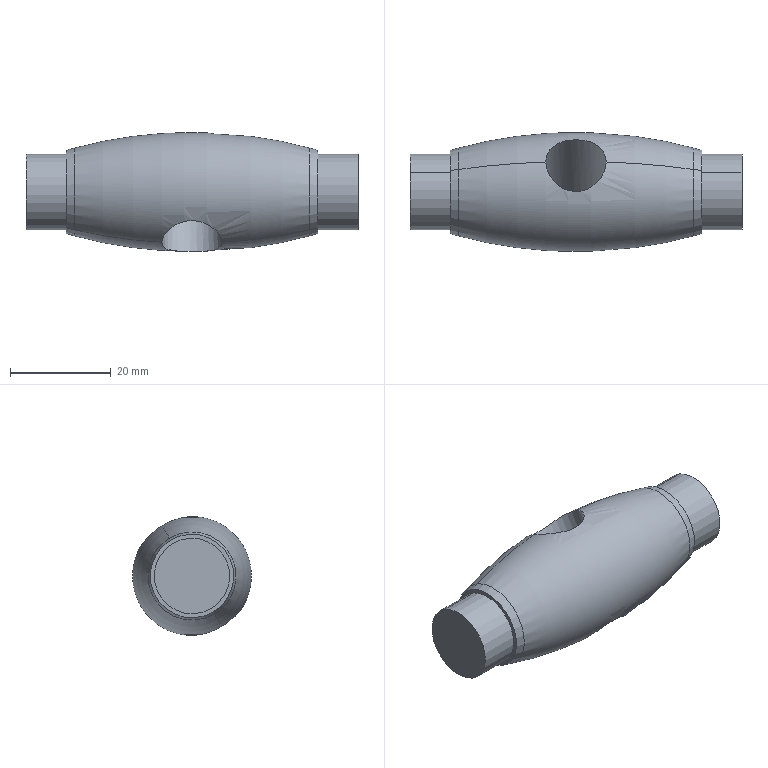Component | SolidWorks | ShaftStop-1 | 1 solid | 16 faces | volume 18258 mm3 | cylinder 6 | cone 4 | plane 4 | torus 2 | commonest cylinder face diameters 15 x4 12 x2
build123d program:
from build123d import *

# Parameters (mm, degrees)
SKETCH1_R           = 15
BOSS_EXTRUDE1_DEPTH = 25
BOSS_EXTRUDE1_TAPER = 15
SKETCH2_R           = 7.5
BOSS_EXTRUDE2_DEPTH = 8
FILLET1_R           = 90
SKETCH3_R           = 6
CUT_EXTRUDE1_DEPTH  = 16.5


with BuildPart() as part:
    # Sketch1 → Boss-Extrude1 (new body)
    with BuildSketch(Plane.XY):
        Circle(SKETCH1_R)
    boss_extrude1 = extrude(amount=BOSS_EXTRUDE1_DEPTH, taper=BOSS_EXTRUDE1_TAPER)

    # Sketch2 → Boss-Extrude2 (add)
    with BuildSketch(Plane.XY.offset(25)):
        Circle(SKETCH2_R)
    boss_extrude2 = extrude(amount=BOSS_EXTRUDE2_DEPTH)

    # Mirror1: Boss-Extrude1, Boss-Extrude2 across plane
    add(boss_extrude1.mirror(Plane.XY))
    add(boss_extrude2.mirror(Plane.XY))

    # Fillet1
    fillet1_edges = [part.edges().sort_by_distance(p)[0] for p in [
        (-15, 0, 0),
    ]]
    fillet(fillet1_edges, radius=FILLET1_R)

    # Sketch3 → Cut-Extrude1 (cut, symmetric)
    with BuildSketch(Plane(origin=(0, 0, 0), x_dir=(0, 0, -1), z_dir=(1, 0, 0))):
        with Locations(Location((0, 0, 0), (0, 0, 299.667))):
            Circle(SKETCH3_R)
    extrude(amount=CUT_EXTRUDE1_DEPTH, both=True, mode=Mode.SUBTRACT)


solid = part.part

# Placed as in the assembly
solid = solid.moved(Location((0, 95, 2.5), (3.838, 90, -34.621)))
STEP:
#1=COLOUR_RGB('',0.7922,0.8196,0.9333);
#2=FILL_AREA_STYLE_COLOUR('',#1);
#3=FILL_AREA_STYLE('',(#2));
#4=SURFACE_STYLE_FILL_AREA(#3);
#5=SURFACE_SIDE_STYLE('',(#4));
#6=SURFACE_STYLE_USAGE(.BOTH.,#5);
#7=PRESENTATION_STYLE_ASSIGNMENT((#6));
#8=CARTESIAN_POINT('',(-0.2362,3.974,0.4916));
#9=VERTEX_POINT('',#8);
#10=CARTESIAN_POINT('',(0.2362,3.974,0.4916));
#11=VERTEX_POINT('',#10);
#12=CARTESIAN_POINT('',(-0.2362,3.974,0.4916));
#13=CARTESIAN_POINT('',(-0.2362,3.961,0.4997));
#14=CARTESIAN_POINT('',(-0.2347,3.947,0.507));
#15=CARTESIAN_POINT('',(-0.23,3.926,0.517));
#16=CARTESIAN_POINT('',(-0.2281,3.919,0.5202));
#17=CARTESIAN_POINT('',(-0.2235,3.906,0.5261));
#18=CARTESIAN_POINT('',(-0.2209,3.899,0.5289));
#19=CARTESIAN_POINT('',(-0.2119,3.878,0.5366));
#20=CARTESIAN_POINT('',(-0.2046,3.865,0.541));
#21=CARTESIAN_POINT('',(-0.1874,3.84,0.5483));
#22=CARTESIAN_POINT('',(-0.1777,3.828,0.5513));
#23=CARTESIAN_POINT('',(-0.1454,3.795,0.5584));
#24=CARTESIAN_POINT('',(-0.1191,3.776,0.5609));
#25=CARTESIAN_POINT('',(-0.07654,3.756,0.563));
#26=CARTESIAN_POINT('',(-0.0617,3.751,0.5634));
#27=CARTESIAN_POINT('',(-0.03086,3.744,0.5639));
#28=CARTESIAN_POINT('',(-0.01535,3.743,0.564));
#29=CARTESIAN_POINT('',(0.01585,3.743,0.564));
#30=CARTESIAN_POINT('',(0.03171,3.744,0.5639));
#31=CARTESIAN_POINT('',(0.06224,3.751,0.5633));
#32=CARTESIAN_POINT('',(0.07702,3.756,0.5629));
#33=CARTESIAN_POINT('',(0.1057,3.769,0.5616));
#34=CARTESIAN_POINT('',(0.1192,3.777,0.5606));
#35=CARTESIAN_POINT('',(0.1445,3.796,0.5578));
#36=CARTESIAN_POINT('',(0.1564,3.806,0.556));
#37=CARTESIAN_POINT('',(0.178,3.828,0.5512));
#38=CARTESIAN_POINT('',(0.1876,3.84,0.5482));
#39=CARTESIAN_POINT('',(0.2047,3.865,0.5409));
#40=CARTESIAN_POINT('',(0.2121,3.879,0.5365));
#41=CARTESIAN_POINT('',(0.2239,3.906,0.5262));
#42=CARTESIAN_POINT('',(0.2285,3.919,0.5204));
#43=CARTESIAN_POINT('',(0.2331,3.94,0.5104));
#44=CARTESIAN_POINT('',(0.2343,3.947,0.5068));
#45=CARTESIAN_POINT('',(0.2358,3.961,0.4994));
#46=CARTESIAN_POINT('',(0.2362,3.968,0.4956));
#47=CARTESIAN_POINT('',(0.2362,3.974,0.4916));
#48=B_SPLINE_CURVE_WITH_KNOTS('',3,(#12,#13,#14,#15,#16,#17,#18,#19,#20,#21,#22,#23,#24,#25,#26,#27,#28,#29,#30,#31,#32,#33,#34,#35,#36,#37,#38,#39,#40,#41,#42,#43,#44,#45,#46,#47),.UNSPECIFIED.,.F.,.F.,(4,2,2,2,2,2,2,2,2,2,2,2,2,2,2,2,2,4),(0.03167,0.03286,0.03346,0.03405,0.03524,0.03643,0.03881,0.04,0.04118,0.04237,0.04356,0.04475,0.04594,0.04713,0.04832,0.04951,0.0501,0.0507),.UNSPECIFIED.);
#49=EDGE_CURVE('',#9,#11,#48,.T.);
#50=ORIENTED_EDGE('',*,*,#49,.T.);
#51=CARTESIAN_POINT('',(0.2362,3.506,-0.2948));
#52=VERTEX_POINT('',#51);
#53=CARTESIAN_POINT('',(0.2362,4.073,0.6565));
#54=DIRECTION('',(0.,-0.5118,-0.8591));
#55=VECTOR('',#54,39.37);
#56=LINE('',#53,#55);
#57=EDGE_CURVE('',#11,#52,#56,.T.);
#58=ORIENTED_EDGE('',*,*,#57,.T.);
#59=CARTESIAN_POINT('',(-0.2362,3.506,-0.2948));
#60=VERTEX_POINT('',#59);
#61=CARTESIAN_POINT('',(0.2362,3.506,-0.2948));
#62=CARTESIAN_POINT('',(0.2362,3.492,-0.2868));
#63=CARTESIAN_POINT('',(0.2346,3.479,-0.278));
#64=CARTESIAN_POINT('',(0.2285,3.454,-0.26));
#65=CARTESIAN_POINT('',(0.2239,3.443,-0.2507));
#66=CARTESIAN_POINT('',(0.2118,3.42,-0.2316));
#67=CARTESIAN_POINT('',(0.2045,3.41,-0.2221));
#68=CARTESIAN_POINT('',(0.1874,3.392,-0.2034));
#69=CARTESIAN_POINT('',(0.1775,3.384,-0.1942));
#70=CARTESIAN_POINT('',(0.1559,3.369,-0.1769));
#71=CARTESIAN_POINT('',(0.1442,3.362,-0.1689));
#72=CARTESIAN_POINT('',(0.1251,3.354,-0.1579));
#73=CARTESIAN_POINT('',(0.1185,3.352,-0.1543));
#74=CARTESIAN_POINT('',(0.1049,3.347,-0.1479));
#75=CARTESIAN_POINT('',(0.09796,3.345,-0.1449));
#76=CARTESIAN_POINT('',(0.07672,3.339,-0.1369));
#77=CARTESIAN_POINT('',(0.06197,3.337,-0.1326));
#78=CARTESIAN_POINT('',(0.03886,3.334,-0.1283));
#79=CARTESIAN_POINT('',(0.03105,3.333,-0.1272));
#80=CARTESIAN_POINT('',(0.01549,3.332,-0.1257));
#81=CARTESIAN_POINT('',(-0.00008135,3.332,-0.125));
#82=CARTESIAN_POINT('',(-0.01568,3.332,-0.1257));
#83=CARTESIAN_POINT('',(-0.0313,3.333,-0.1272));
#84=CARTESIAN_POINT('',(-0.03916,3.334,-0.1283));
#85=CARTESIAN_POINT('',(-0.06217,3.337,-0.1327));
#86=CARTESIAN_POINT('',(-0.07696,3.339,-0.1369));
#87=CARTESIAN_POINT('',(-0.1055,3.347,-0.1478));
#88=CARTESIAN_POINT('',(-0.1193,3.352,-0.1545));
#89=CARTESIAN_POINT('',(-0.1446,3.363,-0.1691));
#90=CARTESIAN_POINT('',(-0.1563,3.369,-0.1772));
#91=CARTESIAN_POINT('',(-0.1779,3.384,-0.1945));
#92=CARTESIAN_POINT('',(-0.1877,3.392,-0.2037));
#93=CARTESIAN_POINT('',(-0.2047,3.411,-0.2223));
#94=CARTESIAN_POINT('',(-0.2119,3.421,-0.2318));
#95=CARTESIAN_POINT('',(-0.2209,3.437,-0.246));
#96=CARTESIAN_POINT('',(-0.2236,3.443,-0.2508));
#97=CARTESIAN_POINT('',(-0.2281,3.455,-0.2601));
#98=CARTESIAN_POINT('',(-0.23,3.461,-0.2647));
#99=CARTESIAN_POINT('',(-0.2331,3.473,-0.2736));
#100=CARTESIAN_POINT('',(-0.2343,3.479,-0.278));
#101=CARTESIAN_POINT('',(-0.2358,3.492,-0.2865));
#102=CARTESIAN_POINT('',(-0.2362,3.499,-0.2907));
#103=CARTESIAN_POINT('',(-0.2362,3.506,-0.2948));
#104=B_SPLINE_CURVE_WITH_KNOTS('',3,(#61,#62,#63,#64,#65,#66,#67,#68,#69,#70,#71,#72,#73,#74,#75,#76,#77,#78,#79,#80,#81,#82,#83,#84,#85,#86,#87,#88,#89,#90,#91,#92,#93,#94,#95,#96,#97,#98,#99,#100,#101,#102,#103),.UNSPECIFIED.,.F.,.F.,(4,2,2,2,2,2,2,2,2,2,1,2,2,2,2,2,2,2,2,2,2,4),(0.02541,0.02659,0.02778,0.02897,0.03016,0.03134,0.03194,0.03253,0.03372,0.03431,0.03491,0.0355,0.03609,0.03728,0.03847,0.03966,0.04084,0.04203,0.04263,0.04322,0.04381,0.04441),.UNSPECIFIED.);
#105=EDGE_CURVE('',#52,#60,#104,.T.);
#106=ORIENTED_EDGE('',*,*,#105,.T.);
#107=CARTESIAN_POINT('',(-0.2362,4.073,0.6565));
#108=DIRECTION('',(0.,-0.5118,-0.8591));
#109=VECTOR('',#108,39.37);
#110=LINE('',#107,#109);
#111=EDGE_CURVE('',#9,#60,#110,.T.);
#112=ORIENTED_EDGE('',*,*,#111,.F.);
#113=EDGE_LOOP('',(#50,#58,#106,#112));
#114=FACE_OUTER_BOUND('',#113,.T.);
#115=CARTESIAN_POINT('',(0.,4.073,0.6565));
#116=DIRECTION('',(0.,-0.5118,-0.8591));
#117=DIRECTION('',(-1.,0.,0.));
#118=AXIS2_PLACEMENT_3D('',#115,#116,#117);
#119=CYLINDRICAL_SURFACE('',#118,0.2362);
#120=ADVANCED_FACE('',(#114),#119,.F.);
#121=CARTESIAN_POINT('',(0.9171,3.564,-0.1978));
#122=VERTEX_POINT('',#121);
#123=CARTESIAN_POINT('',(0.9171,3.917,0.3947));
#124=VERTEX_POINT('',#123);
#125=CARTESIAN_POINT('',(0.9171,3.74,0.09843));
#126=DIRECTION('',(1.,0.,0.));
#127=DIRECTION('',(0.,0.5118,0.8591));
#128=AXIS2_PLACEMENT_3D('',#125,#126,#127);
#129=CIRCLE('',#128,0.3448);
#130=EDGE_CURVE('',#122,#124,#129,.T.);
#131=ORIENTED_EDGE('',*,*,#130,.F.);
#132=CARTESIAN_POINT('',(0.,5.315,2.743));
#133=DIRECTION('',(0.,0.8591,-0.5118));
#134=DIRECTION('',(0.,0.5118,0.8591));
#135=AXIS2_PLACEMENT_3D('',#132,#133,#134);
#136=CIRCLE('',#135,3.543);
#137=EDGE_CURVE('',#122,#52,#136,.T.);
#138=ORIENTED_EDGE('',*,*,#137,.T.);
#139=CARTESIAN_POINT('',(-0.2362,3.506,-0.2948));
#140=CARTESIAN_POINT('',(-0.2362,3.519,-0.3028));
#141=CARTESIAN_POINT('',(-0.2347,3.533,-0.3102));
#142=CARTESIAN_POINT('',(-0.2285,3.561,-0.3235));
#143=CARTESIAN_POINT('',(-0.2239,3.575,-0.3295));
#144=CARTESIAN_POINT('',(-0.2119,3.602,-0.3397));
#145=CARTESIAN_POINT('',(-0.2046,3.615,-0.3441));
#146=CARTESIAN_POINT('',(-0.1874,3.641,-0.3515));
#147=CARTESIAN_POINT('',(-0.1777,3.652,-0.3544));
#148=CARTESIAN_POINT('',(-0.1615,3.669,-0.358));
#149=CARTESIAN_POINT('',(-0.1559,3.674,-0.359));
#150=CARTESIAN_POINT('',(-0.144,3.685,-0.3609));
#151=CARTESIAN_POINT('',(-0.1378,3.69,-0.3617));
#152=CARTESIAN_POINT('',(-0.1188,3.703,-0.3638));
#153=CARTESIAN_POINT('',(-0.1053,3.711,-0.3647));
#154=CARTESIAN_POINT('',(-0.07694,3.724,-0.3661));
#155=CARTESIAN_POINT('',(-0.06182,3.729,-0.3665));
#156=CARTESIAN_POINT('',(-0.03136,3.736,-0.367));
#157=CARTESIAN_POINT('',(-0.01589,3.738,-0.3671));
#158=CARTESIAN_POINT('',(0.007708,3.738,-0.3671));
#159=CARTESIAN_POINT('',(0.01566,3.737,-0.3671));
#160=CARTESIAN_POINT('',(0.03126,3.736,-0.367));
#161=CARTESIAN_POINT('',(0.04669,3.733,-0.3668));
#162=CARTESIAN_POINT('',(0.06175,3.729,-0.3665));
#163=CARTESIAN_POINT('',(0.07664,3.724,-0.366));
#164=CARTESIAN_POINT('',(0.08402,3.721,-0.3657));
#165=CARTESIAN_POINT('',(0.1054,3.711,-0.3647));
#166=CARTESIAN_POINT('',(0.1189,3.703,-0.3638));
#167=CARTESIAN_POINT('',(0.138,3.689,-0.3617));
#168=CARTESIAN_POINT('',(0.1442,3.684,-0.3609));
#169=CARTESIAN_POINT('',(0.156,3.674,-0.359));
#170=CARTESIAN_POINT('',(0.1617,3.669,-0.358));
#171=CARTESIAN_POINT('',(0.1778,3.652,-0.3544));
#172=CARTESIAN_POINT('',(0.1875,3.64,-0.3514));
#173=CARTESIAN_POINT('',(0.2047,3.615,-0.344));
#174=CARTESIAN_POINT('',(0.212,3.602,-0.3397));
#175=CARTESIAN_POINT('',(0.2209,3.582,-0.332));
#176=CARTESIAN_POINT('',(0.2235,3.575,-0.3293));
#177=CARTESIAN_POINT('',(0.2281,3.561,-0.3233));
#178=CARTESIAN_POINT('',(0.2301,3.554,-0.3201));
#179=CARTESIAN_POINT('',(0.2347,3.533,-0.3101));
#180=CARTESIAN_POINT('',(0.2362,3.519,-0.3028));
#181=CARTESIAN_POINT('',(0.2362,3.506,-0.2948));
#182=B_SPLINE_CURVE_WITH_KNOTS('',3,(#139,#140,#141,#142,#143,#144,#145,#146,#147,#148,#149,#150,#151,#152,#153,#154,#155,#156,#157,#158,#159,#160,#161,#162,#163,#164,#165,#166,#167,#168,#169,#170,#171,#172,#173,#174,#175,#176,#177,#178,#179,#180,#181),.UNSPECIFIED.,.F.,.F.,(4,2,2,2,2,2,2,2,2,2,2,1,2,2,2,2,2,2,2,2,2,4),(0.006395,0.007583,0.008771,0.009959,0.01115,0.01174,0.01234,0.01352,0.01471,0.0159,0.01649,0.01709,0.01768,0.01828,0.01947,0.02006,0.02065,0.02184,0.02303,0.02362,0.02422,0.02541),.UNSPECIFIED.);
#183=EDGE_CURVE('',#60,#52,#182,.T.);
#184=ORIENTED_EDGE('',*,*,#183,.F.);
#185=CARTESIAN_POINT('',(-0.9171,3.564,-0.1978));
#186=VERTEX_POINT('',#185);
#187=CARTESIAN_POINT('',(0.,5.315,2.743));
#188=DIRECTION('',(0.,0.8591,-0.5118));
#189=DIRECTION('',(0.,0.5118,0.8591));
#190=AXIS2_PLACEMENT_3D('',#187,#188,#189);
#191=CIRCLE('',#190,3.543);
#192=EDGE_CURVE('',#60,#186,#191,.T.);
#193=ORIENTED_EDGE('',*,*,#192,.T.);
#194=CARTESIAN_POINT('',(-0.9171,3.917,0.3947));
#195=VERTEX_POINT('',#194);
#196=CARTESIAN_POINT('',(-0.9171,3.74,0.09843));
#197=DIRECTION('',(-1.,0.,0.));
#198=DIRECTION('',(0.,-0.5118,-0.8591));
#199=AXIS2_PLACEMENT_3D('',#196,#197,#198);
#200=CIRCLE('',#199,0.3448);
#201=EDGE_CURVE('',#195,#186,#200,.T.);
#202=ORIENTED_EDGE('',*,*,#201,.F.);
#203=CARTESIAN_POINT('',(0.,2.165,-2.546));
#204=DIRECTION('',(0.,-0.8591,0.5118));
#205=DIRECTION('',(0.,-0.5118,-0.8591));
#206=AXIS2_PLACEMENT_3D('',#203,#204,#205);
#207=CIRCLE('',#206,3.543);
#208=EDGE_CURVE('',#9,#195,#207,.T.);
#209=ORIENTED_EDGE('',*,*,#208,.F.);
#210=CARTESIAN_POINT('',(0.2362,3.974,0.4916));
#211=CARTESIAN_POINT('',(0.2362,3.981,0.4876));
#212=CARTESIAN_POINT('',(0.2358,3.988,0.4835));
#213=CARTESIAN_POINT('',(0.2343,4.001,0.4749));
#214=CARTESIAN_POINT('',(0.2331,4.007,0.4705));
#215=CARTESIAN_POINT('',(0.2285,4.026,0.4569));
#216=CARTESIAN_POINT('',(0.2239,4.038,0.4476));
#217=CARTESIAN_POINT('',(0.212,4.06,0.4287));
#218=CARTESIAN_POINT('',(0.2045,4.07,0.419));
#219=CARTESIAN_POINT('',(0.1875,4.088,0.4003));
#220=CARTESIAN_POINT('',(0.1778,4.097,0.3912));
#221=CARTESIAN_POINT('',(0.156,4.111,0.3738));
#222=CARTESIAN_POINT('',(0.1442,4.118,0.3657));
#223=CARTESIAN_POINT('',(0.1253,4.126,0.3548));
#224=CARTESIAN_POINT('',(0.1187,4.129,0.3513));
#225=CARTESIAN_POINT('',(0.1052,4.133,0.3449));
#226=CARTESIAN_POINT('',(0.09814,4.135,0.3419));
#227=CARTESIAN_POINT('',(0.07676,4.141,0.3337));
#228=CARTESIAN_POINT('',(0.06204,4.144,0.3295));
#229=CARTESIAN_POINT('',(0.03159,4.147,0.3237));
#230=CARTESIAN_POINT('',(0.01569,4.148,0.3222));
#231=CARTESIAN_POINT('',(-0.01557,4.148,0.3222));
#232=CARTESIAN_POINT('',(-0.03108,4.148,0.3237));
#233=CARTESIAN_POINT('',(-0.06188,4.144,0.3295));
#234=CARTESIAN_POINT('',(-0.07681,4.141,0.3338));
#235=CARTESIAN_POINT('',(-0.1052,4.134,0.3445));
#236=CARTESIAN_POINT('',(-0.119,4.129,0.3511));
#237=CARTESIAN_POINT('',(-0.1444,4.118,0.3658));
#238=CARTESIAN_POINT('',(-0.1561,4.111,0.3739));
#239=CARTESIAN_POINT('',(-0.1723,4.1,0.3869));
#240=CARTESIAN_POINT('',(-0.1775,4.096,0.3914));
#241=CARTESIAN_POINT('',(-0.1873,4.088,0.4005));
#242=CARTESIAN_POINT('',(-0.1918,4.084,0.4051));
#243=CARTESIAN_POINT('',(-0.2046,4.07,0.4191));
#244=CARTESIAN_POINT('',(-0.2119,4.06,0.4285));
#245=CARTESIAN_POINT('',(-0.2239,4.038,0.4476));
#246=CARTESIAN_POINT('',(-0.2285,4.026,0.457));
#247=CARTESIAN_POINT('',(-0.2331,4.007,0.4704));
#248=CARTESIAN_POINT('',(-0.2343,4.001,0.4748));
#249=CARTESIAN_POINT('',(-0.2358,3.988,0.4834));
#250=CARTESIAN_POINT('',(-0.2362,3.981,0.4876));
#251=CARTESIAN_POINT('',(-0.2362,3.974,0.4916));
#252=B_SPLINE_CURVE_WITH_KNOTS('',3,(#210,#211,#212,#213,#214,#215,#216,#217,#218,#219,#220,#221,#222,#223,#224,#225,#226,#227,#228,#229,#230,#231,#232,#233,#234,#235,#236,#237,#238,#239,#240,#241,#242,#243,#244,#245,#246,#247,#248,#249,#250,#251),.UNSPECIFIED.,.F.,.F.,(4,2,2,2,2,2,2,2,2,2,2,2,2,2,2,2,2,2,2,2,4),(0.01264,0.01324,0.01383,0.01502,0.01621,0.0174,0.01859,0.01918,0.01978,0.02097,0.02216,0.02335,0.02454,0.02572,0.02691,0.02751,0.0281,0.02929,0.03048,0.03108,0.03167),.UNSPECIFIED.);
#253=EDGE_CURVE('',#11,#9,#252,.T.);
#254=ORIENTED_EDGE('',*,*,#253,.F.);
#255=CARTESIAN_POINT('',(0.,2.165,-2.546));
#256=DIRECTION('',(0.,-0.8591,0.5118));
#257=DIRECTION('',(0.,-0.5118,-0.8591));
#258=AXIS2_PLACEMENT_3D('',#255,#256,#257);
#259=CIRCLE('',#258,3.543);
#260=EDGE_CURVE('',#124,#11,#259,.T.);
#261=ORIENTED_EDGE('',*,*,#260,.F.);
#262=EDGE_LOOP('',(#131,#138,#184,#193,#202,#209,#254,#261));
#263=FACE_OUTER_BOUND('',#262,.T.);
#264=CARTESIAN_POINT('',(0.,3.74,0.09843));
#265=DIRECTION('',(-1.,0.,0.));
#266=DIRECTION('',(0.,0.5118,0.8591));
#267=AXIS2_PLACEMENT_3D('',#264,#265,#266);
#268=TOROIDAL_SURFACE('',#267,-3.078,3.543);
#269=ADVANCED_FACE('',(#263),#268,.T.);
#270=CARTESIAN_POINT('',(-1.299,3.589,-0.1553));
#271=VERTEX_POINT('',#270);
#272=CARTESIAN_POINT('',(-1.299,3.891,0.3521));
#273=VERTEX_POINT('',#272);
#274=CARTESIAN_POINT('',(-1.299,3.74,0.09843));
#275=DIRECTION('',(1.,0.,0.));
#276=DIRECTION('',(0.,-0.5118,-0.8591));
#277=AXIS2_PLACEMENT_3D('',#274,#275,#276);
#278=CIRCLE('',#277,0.2953);
#279=EDGE_CURVE('',#271,#273,#278,.T.);
#280=ORIENTED_EDGE('',*,*,#279,.T.);
#281=CARTESIAN_POINT('',(-0.9843,3.891,0.3521));
#282=VERTEX_POINT('',#281);
#283=CARTESIAN_POINT('',(-1.299,3.891,0.3521));
#284=DIRECTION('',(1.,0.,0.));
#285=VECTOR('',#284,39.37);
#286=LINE('',#283,#285);
#287=EDGE_CURVE('',#273,#282,#286,.T.);
#288=ORIENTED_EDGE('',*,*,#287,.T.);
#289=CARTESIAN_POINT('',(-0.9843,3.589,-0.1553));
#290=VERTEX_POINT('',#289);
#291=CARTESIAN_POINT('',(-0.9843,3.74,0.09843));
#292=DIRECTION('',(-1.,0.,0.));
#293=DIRECTION('',(0.,0.5118,0.8591));
#294=AXIS2_PLACEMENT_3D('',#291,#292,#293);
#295=CIRCLE('',#294,0.2953);
#296=EDGE_CURVE('',#282,#290,#295,.T.);
#297=ORIENTED_EDGE('',*,*,#296,.T.);
#298=CARTESIAN_POINT('',(-1.299,3.589,-0.1553));
#299=DIRECTION('',(1.,0.,0.));
#300=VECTOR('',#299,39.37);
#301=LINE('',#298,#300);
#302=EDGE_CURVE('',#271,#290,#301,.T.);
#303=ORIENTED_EDGE('',*,*,#302,.F.);
#304=EDGE_LOOP('',(#280,#288,#297,#303));
#305=FACE_OUTER_BOUND('',#304,.T.);
#306=CARTESIAN_POINT('',(-1.299,3.74,0.09843));
#307=DIRECTION('',(1.,0.,0.));
#308=DIRECTION('',(0.,-0.5118,-0.8591));
#309=AXIS2_PLACEMENT_3D('',#306,#307,#308);
#310=CYLINDRICAL_SURFACE('',#309,0.2953);
#311=ADVANCED_FACE('',(#305),#310,.T.);
#312=CARTESIAN_POINT('',(-0.9843,3.573,-0.1824));
#313=VERTEX_POINT('',#312);
#314=CARTESIAN_POINT('',(-0.9843,3.907,0.3792));
#315=VERTEX_POINT('',#314);
#316=CARTESIAN_POINT('',(-0.9843,3.74,0.09843));
#317=DIRECTION('',(1.,0.,0.));
#318=DIRECTION('',(0.,0.5118,0.8591));
#319=AXIS2_PLACEMENT_3D('',#316,#317,#318);
#320=CIRCLE('',#319,0.3268);
#321=EDGE_CURVE('',#313,#315,#320,.T.);
#322=ORIENTED_EDGE('',*,*,#321,.T.);
#323=CARTESIAN_POINT('',(0.,4.042,0.6058));
#324=DIRECTION('',(0.9659,0.1325,0.2224));
#325=VECTOR('',#324,39.37);
#326=LINE('',#323,#325);
#327=EDGE_CURVE('',#315,#195,#326,.T.);
#328=ORIENTED_EDGE('',*,*,#327,.T.);
#329=ORIENTED_EDGE('',*,*,#201,.T.);
#330=CARTESIAN_POINT('',(0.,3.438,-0.4089));
#331=DIRECTION('',(0.9659,-0.1325,-0.2224));
#332=VECTOR('',#331,39.37);
#333=LINE('',#330,#332);
#334=EDGE_CURVE('',#313,#186,#333,.T.);
#335=ORIENTED_EDGE('',*,*,#334,.F.);
#336=EDGE_LOOP('',(#322,#328,#329,#335));
#337=FACE_OUTER_BOUND('',#336,.T.);
#338=CARTESIAN_POINT('',(0.,3.74,0.09843));
#339=DIRECTION('',(1.,0.,0.));
#340=DIRECTION('',(0.,-0.5118,-0.8591));
#341=AXIS2_PLACEMENT_3D('',#338,#339,#340);
#342=CONICAL_SURFACE('',#341,0.5906,0.2618);
#343=ADVANCED_FACE('',(#337),#342,.T.);
#344=CARTESIAN_POINT('',(1.299,3.589,-0.1553));
#345=VERTEX_POINT('',#344);
#346=CARTESIAN_POINT('',(1.299,3.891,0.3521));
#347=VERTEX_POINT('',#346);
#348=CARTESIAN_POINT('',(1.299,3.74,0.09843));
#349=DIRECTION('',(1.,0.,0.));
#350=DIRECTION('',(0.,-0.5118,-0.8591));
#351=AXIS2_PLACEMENT_3D('',#348,#349,#350);
#352=CIRCLE('',#351,0.2953);
#353=EDGE_CURVE('',#345,#347,#352,.T.);
#354=ORIENTED_EDGE('',*,*,#353,.F.);
#355=CARTESIAN_POINT('',(0.9843,3.589,-0.1553));
#356=VERTEX_POINT('',#355);
#357=CARTESIAN_POINT('',(1.299,3.589,-0.1553));
#358=DIRECTION('',(-1.,0.,0.));
#359=VECTOR('',#358,39.37);
#360=LINE('',#357,#359);
#361=EDGE_CURVE('',#345,#356,#360,.T.);
#362=ORIENTED_EDGE('',*,*,#361,.T.);
#363=CARTESIAN_POINT('',(0.9843,3.891,0.3521));
#364=VERTEX_POINT('',#363);
#365=CARTESIAN_POINT('',(0.9843,3.74,0.09843));
#366=DIRECTION('',(1.,0.,0.));
#367=DIRECTION('',(0.,-0.5118,-0.8591));
#368=AXIS2_PLACEMENT_3D('',#365,#366,#367);
#369=CIRCLE('',#368,0.2953);
#370=EDGE_CURVE('',#356,#364,#369,.T.);
#371=ORIENTED_EDGE('',*,*,#370,.T.);
#372=CARTESIAN_POINT('',(1.299,3.891,0.3521));
#373=DIRECTION('',(-1.,0.,0.));
#374=VECTOR('',#373,39.37);
#375=LINE('',#372,#374);
#376=EDGE_CURVE('',#347,#364,#375,.T.);
#377=ORIENTED_EDGE('',*,*,#376,.F.);
#378=EDGE_LOOP('',(#354,#362,#371,#377));
#379=FACE_OUTER_BOUND('',#378,.T.);
#380=CARTESIAN_POINT('',(1.299,3.74,0.09843));
#381=DIRECTION('',(-1.,0.,0.));
#382=DIRECTION('',(0.,0.5118,0.8591));
#383=AXIS2_PLACEMENT_3D('',#380,#381,#382);
#384=CYLINDRICAL_SURFACE('',#383,0.2953);
#385=ADVANCED_FACE('',(#379),#384,.T.);
#386=CARTESIAN_POINT('',(0.9843,3.907,0.3792));
#387=VERTEX_POINT('',#386);
#388=CARTESIAN_POINT('',(0.9843,3.573,-0.1824));
#389=VERTEX_POINT('',#388);
#390=CARTESIAN_POINT('',(0.9843,3.74,0.09843));
#391=DIRECTION('',(1.,0.,0.));
#392=DIRECTION('',(0.,-0.5118,-0.8591));
#393=AXIS2_PLACEMENT_3D('',#390,#391,#392);
#394=CIRCLE('',#393,0.3268);
#395=EDGE_CURVE('',#387,#389,#394,.T.);
#396=ORIENTED_EDGE('',*,*,#395,.F.);
#397=CARTESIAN_POINT('',(0.,4.042,0.6058));
#398=DIRECTION('',(-0.9659,0.1325,0.2224));
#399=VECTOR('',#398,39.37);
#400=LINE('',#397,#399);
#401=EDGE_CURVE('',#387,#124,#400,.T.);
#402=ORIENTED_EDGE('',*,*,#401,.T.);
#403=CARTESIAN_POINT('',(0.9171,3.74,0.09843));
#404=DIRECTION('',(1.,0.,0.));
#405=DIRECTION('',(0.,0.5118,0.8591));
#406=AXIS2_PLACEMENT_3D('',#403,#404,#405);
#407=CIRCLE('',#406,0.3448);
#408=EDGE_CURVE('',#124,#122,#407,.T.);
#409=ORIENTED_EDGE('',*,*,#408,.T.);
#410=CARTESIAN_POINT('',(0.,3.438,-0.4089));
#411=DIRECTION('',(-0.9659,-0.1325,-0.2224));
#412=VECTOR('',#411,39.37);
#413=LINE('',#410,#412);
#414=EDGE_CURVE('',#389,#122,#413,.T.);
#415=ORIENTED_EDGE('',*,*,#414,.F.);
#416=EDGE_LOOP('',(#396,#402,#409,#415));
#417=FACE_OUTER_BOUND('',#416,.T.);
#418=CARTESIAN_POINT('',(0.,3.74,0.09843));
#419=DIRECTION('',(-1.,0.,0.));
#420=DIRECTION('',(0.,-0.5118,-0.8591));
#421=AXIS2_PLACEMENT_3D('',#418,#419,#420);
#422=CONICAL_SURFACE('',#421,0.5906,0.2618);
#423=ADVANCED_FACE('',(#417),#422,.T.);
#424=CARTESIAN_POINT('',(0.9843,3.74,0.09843));
#425=DIRECTION('',(1.,0.,0.));
#426=DIRECTION('',(0.,-0.5118,-0.8591));
#427=AXIS2_PLACEMENT_3D('',#424,#425,#426);
#428=CIRCLE('',#427,0.3268);
#429=EDGE_CURVE('',#389,#387,#428,.T.);
#430=ORIENTED_EDGE('',*,*,#429,.T.);
#431=ORIENTED_EDGE('',*,*,#395,.T.);
#432=EDGE_LOOP('',(#430,#431));
#433=FACE_OUTER_BOUND('',#432,.T.);
#434=CARTESIAN_POINT('',(0.9843,3.74,0.09843));
#435=DIRECTION('',(1.,0.,0.));
#436=DIRECTION('',(0.,-0.5118,-0.8591));
#437=AXIS2_PLACEMENT_3D('',#434,#435,#436);
#438=CIRCLE('',#437,0.2953);
#439=EDGE_CURVE('',#364,#356,#438,.T.);
#440=ORIENTED_EDGE('',*,*,#439,.F.);
#441=ORIENTED_EDGE('',*,*,#370,.F.);
#442=EDGE_LOOP('',(#440,#441));
#443=FACE_BOUND('',#442,.T.);
#444=CARTESIAN_POINT('',(0.9843,3.74,0.09843));
#445=DIRECTION('',(1.,0.,0.));
#446=DIRECTION('',(0.,-0.5118,-0.8591));
#447=AXIS2_PLACEMENT_3D('',#444,#445,#446);
#448=PLANE('',#447);
#449=ADVANCED_FACE('',(#433,#443),#448,.T.);
#450=ORIENTED_EDGE('',*,*,#401,.F.);
#451=ORIENTED_EDGE('',*,*,#429,.F.);
#452=ORIENTED_EDGE('',*,*,#414,.T.);
#453=ORIENTED_EDGE('',*,*,#130,.T.);
#454=EDGE_LOOP('',(#450,#451,#452,#453));
#455=FACE_OUTER_BOUND('',#454,.T.);
#456=CARTESIAN_POINT('',(0.,3.74,0.09843));
#457=DIRECTION('',(-1.,0.,0.));
#458=DIRECTION('',(0.,-0.5118,-0.8591));
#459=AXIS2_PLACEMENT_3D('',#456,#457,#458);
#460=CONICAL_SURFACE('',#459,0.5906,0.2618);
#461=ADVANCED_FACE('',(#455),#460,.T.);
#462=ORIENTED_EDGE('',*,*,#361,.F.);
#463=CARTESIAN_POINT('',(1.299,3.74,0.09843));
#464=DIRECTION('',(1.,0.,0.));
#465=DIRECTION('',(0.,-0.5118,-0.8591));
#466=AXIS2_PLACEMENT_3D('',#463,#464,#465);
#467=CIRCLE('',#466,0.2953);
#468=EDGE_CURVE('',#347,#345,#467,.T.);
#469=ORIENTED_EDGE('',*,*,#468,.F.);
#470=ORIENTED_EDGE('',*,*,#376,.T.);
#471=ORIENTED_EDGE('',*,*,#439,.T.);
#472=EDGE_LOOP('',(#462,#469,#470,#471));
#473=FACE_OUTER_BOUND('',#472,.T.);
#474=CARTESIAN_POINT('',(1.299,3.74,0.09843));
#475=DIRECTION('',(-1.,0.,0.));
#476=DIRECTION('',(0.,0.5118,0.8591));
#477=AXIS2_PLACEMENT_3D('',#474,#475,#476);
#478=CYLINDRICAL_SURFACE('',#477,0.2953);
#479=ADVANCED_FACE('',(#473),#478,.T.);
#480=ORIENTED_EDGE('',*,*,#468,.T.);
#481=ORIENTED_EDGE('',*,*,#353,.T.);
#482=EDGE_LOOP('',(#480,#481));
#483=FACE_OUTER_BOUND('',#482,.T.);
#484=CARTESIAN_POINT('',(1.299,3.74,0.09843));
#485=DIRECTION('',(1.,0.,0.));
#486=DIRECTION('',(0.,-0.5118,-0.8591));
#487=AXIS2_PLACEMENT_3D('',#484,#485,#486);
#488=PLANE('',#487);
#489=ADVANCED_FACE('',(#483),#488,.T.);
#490=ORIENTED_EDGE('',*,*,#327,.F.);
#491=CARTESIAN_POINT('',(-0.9843,3.74,0.09843));
#492=DIRECTION('',(1.,0.,0.));
#493=DIRECTION('',(0.,0.5118,0.8591));
#494=AXIS2_PLACEMENT_3D('',#491,#492,#493);
#495=CIRCLE('',#494,0.3268);
#496=EDGE_CURVE('',#315,#313,#495,.T.);
#497=ORIENTED_EDGE('',*,*,#496,.T.);
#498=ORIENTED_EDGE('',*,*,#334,.T.);
#499=CARTESIAN_POINT('',(-0.9171,3.74,0.09843));
#500=DIRECTION('',(-1.,0.,0.));
#501=DIRECTION('',(0.,-0.5118,-0.8591));
#502=AXIS2_PLACEMENT_3D('',#499,#500,#501);
#503=CIRCLE('',#502,0.3448);
#504=EDGE_CURVE('',#186,#195,#503,.T.);
#505=ORIENTED_EDGE('',*,*,#504,.T.);
#506=EDGE_LOOP('',(#490,#497,#498,#505));
#507=FACE_OUTER_BOUND('',#506,.T.);
#508=CARTESIAN_POINT('',(0.,3.74,0.09843));
#509=DIRECTION('',(1.,0.,0.));
#510=DIRECTION('',(0.,-0.5118,-0.8591));
#511=AXIS2_PLACEMENT_3D('',#508,#509,#510);
#512=CONICAL_SURFACE('',#511,0.5906,0.2618);
#513=ADVANCED_FACE('',(#507),#512,.T.);
#514=CARTESIAN_POINT('',(-0.9843,3.74,0.09843));
#515=DIRECTION('',(-1.,0.,0.));
#516=DIRECTION('',(0.,0.5118,0.8591));
#517=AXIS2_PLACEMENT_3D('',#514,#515,#516);
#518=CIRCLE('',#517,0.2953);
#519=EDGE_CURVE('',#290,#282,#518,.T.);
#520=ORIENTED_EDGE('',*,*,#519,.F.);
#521=ORIENTED_EDGE('',*,*,#296,.F.);
#522=EDGE_LOOP('',(#520,#521));
#523=FACE_BOUND('',#522,.T.);
#524=ORIENTED_EDGE('',*,*,#321,.F.);
#525=ORIENTED_EDGE('',*,*,#496,.F.);
#526=EDGE_LOOP('',(#524,#525));
#527=FACE_OUTER_BOUND('',#526,.T.);
#528=CARTESIAN_POINT('',(-0.9843,3.74,0.09843));
#529=DIRECTION('',(-1.,0.,0.));
#530=DIRECTION('',(0.,-0.5118,-0.8591));
#531=AXIS2_PLACEMENT_3D('',#528,#529,#530);
#532=PLANE('',#531);
#533=ADVANCED_FACE('',(#523,#527),#532,.T.);
#534=ORIENTED_EDGE('',*,*,#287,.F.);
#535=CARTESIAN_POINT('',(-1.299,3.74,0.09843));
#536=DIRECTION('',(1.,0.,0.));
#537=DIRECTION('',(0.,-0.5118,-0.8591));
#538=AXIS2_PLACEMENT_3D('',#535,#536,#537);
#539=CIRCLE('',#538,0.2953);
#540=EDGE_CURVE('',#273,#271,#539,.T.);
#541=ORIENTED_EDGE('',*,*,#540,.T.);
#542=ORIENTED_EDGE('',*,*,#302,.T.);
#543=ORIENTED_EDGE('',*,*,#519,.T.);
#544=EDGE_LOOP('',(#534,#541,#542,#543));
#545=FACE_OUTER_BOUND('',#544,.T.);
#546=CARTESIAN_POINT('',(-1.299,3.74,0.09843));
#547=DIRECTION('',(1.,0.,0.));
#548=DIRECTION('',(0.,-0.5118,-0.8591));
#549=AXIS2_PLACEMENT_3D('',#546,#547,#548);
#550=CYLINDRICAL_SURFACE('',#549,0.2953);
#551=ADVANCED_FACE('',(#545),#550,.T.);
#552=ORIENTED_EDGE('',*,*,#279,.F.);
#553=ORIENTED_EDGE('',*,*,#540,.F.);
#554=EDGE_LOOP('',(#552,#553));
#555=FACE_OUTER_BOUND('',#554,.T.);
#556=CARTESIAN_POINT('',(-1.299,3.74,0.09843));
#557=DIRECTION('',(-1.,0.,0.));
#558=DIRECTION('',(0.,-0.5118,-0.8591));
#559=AXIS2_PLACEMENT_3D('',#556,#557,#558);
#560=PLANE('',#559);
#561=ADVANCED_FACE('',(#555),#560,.T.);
#562=ORIENTED_EDGE('',*,*,#137,.F.);
#563=ORIENTED_EDGE('',*,*,#408,.F.);
#564=ORIENTED_EDGE('',*,*,#260,.T.);
#565=ORIENTED_EDGE('',*,*,#49,.F.);
#566=ORIENTED_EDGE('',*,*,#208,.T.);
#567=ORIENTED_EDGE('',*,*,#504,.F.);
#568=ORIENTED_EDGE('',*,*,#192,.F.);
#569=ORIENTED_EDGE('',*,*,#105,.F.);
#570=EDGE_LOOP('',(#562,#563,#564,#565,#566,#567,#568,#569));
#571=FACE_OUTER_BOUND('',#570,.T.);
#572=CARTESIAN_POINT('',(0.,3.74,0.09843));
#573=DIRECTION('',(-1.,0.,0.));
#574=DIRECTION('',(0.,0.5118,0.8591));
#575=AXIS2_PLACEMENT_3D('',#572,#573,#574);
#576=TOROIDAL_SURFACE('',#575,-3.078,3.543);
#577=ADVANCED_FACE('',(#571),#576,.T.);
#578=ORIENTED_EDGE('',*,*,#57,.F.);
#579=ORIENTED_EDGE('',*,*,#253,.T.);
#580=ORIENTED_EDGE('',*,*,#111,.T.);
#581=ORIENTED_EDGE('',*,*,#183,.T.);
#582=EDGE_LOOP('',(#578,#579,#580,#581));
#583=FACE_OUTER_BOUND('',#582,.T.);
#584=CARTESIAN_POINT('',(0.,4.073,0.6565));
#585=DIRECTION('',(0.,-0.5118,-0.8591));
#586=DIRECTION('',(-1.,0.,0.));
#587=AXIS2_PLACEMENT_3D('',#584,#585,#586);
#588=CYLINDRICAL_SURFACE('',#587,0.2362);
#589=ADVANCED_FACE('',(#583),#588,.F.);
#590=CLOSED_SHELL('',(#120,#269,#311,#343,#385,#423,#449,#461,#479,#489,#513,#533,#551,#561,#577,#589));
#591=MANIFOLD_SOLID_BREP('',#590);
#592=STYLED_ITEM('',(#7),#591);
#593=PRESENTATION_LAYER_ASSIGNMENT('','',(#592));
#594=(LENGTH_UNIT()NAMED_UNIT(*)SI_UNIT($,.METRE.));
#595=LENGTH_MEASURE_WITH_UNIT(LENGTH_MEASURE(0.0254),#594);
#596=DIMENSIONAL_EXPONENTS(1.,0.,0.,0.,0.,0.,0.);
#597=(CONVERSION_BASED_UNIT('',#595)LENGTH_UNIT()NAMED_UNIT(#596));
#598=UNCERTAINTY_MEASURE_WITH_UNIT(LENGTH_MEASURE(0.00001),#597,'','');
#599=(NAMED_UNIT(*)PLANE_ANGLE_UNIT()SI_UNIT($,.RADIAN.));
#600=(NAMED_UNIT(*)SI_UNIT($,.STERADIAN.)SOLID_ANGLE_UNIT());
#601=(GEOMETRIC_REPRESENTATION_CONTEXT(3)GLOBAL_UNCERTAINTY_ASSIGNED_CONTEXT((#598))GLOBAL_UNIT_ASSIGNED_CONTEXT((#597,#599,#600))REPRESENTATION_CONTEXT('',''));
#602=MECHANICAL_DESIGN_GEOMETRIC_PRESENTATION_REPRESENTATION('',(#592),#601);
#603=CARTESIAN_POINT('',(0.,0.,0.));
#604=DIRECTION('',(0.,0.,1.));
#605=DIRECTION('',(1.,0.,0.));
#606=AXIS2_PLACEMENT_3D('',#603,#604,#605);
#607=(LENGTH_UNIT()NAMED_UNIT(*)SI_UNIT($,.METRE.));
#608=LENGTH_MEASURE_WITH_UNIT(LENGTH_MEASURE(0.0254),#607);
#609=DIMENSIONAL_EXPONENTS(1.,0.,0.,0.,0.,0.,0.);
#610=(CONVERSION_BASED_UNIT('',#608)LENGTH_UNIT()NAMED_UNIT(#609));
#611=UNCERTAINTY_MEASURE_WITH_UNIT(LENGTH_MEASURE(0.00001),#610,'','');
#612=(NAMED_UNIT(*)PLANE_ANGLE_UNIT()SI_UNIT($,.RADIAN.));
#613=(NAMED_UNIT(*)SI_UNIT($,.STERADIAN.)SOLID_ANGLE_UNIT());
#614=(GEOMETRIC_REPRESENTATION_CONTEXT(3)GLOBAL_UNCERTAINTY_ASSIGNED_CONTEXT((#611))GLOBAL_UNIT_ASSIGNED_CONTEXT((#610,#612,#613))REPRESENTATION_CONTEXT('',''));
#615=ADVANCED_BREP_SHAPE_REPRESENTATION('',(#591,#606),#614);